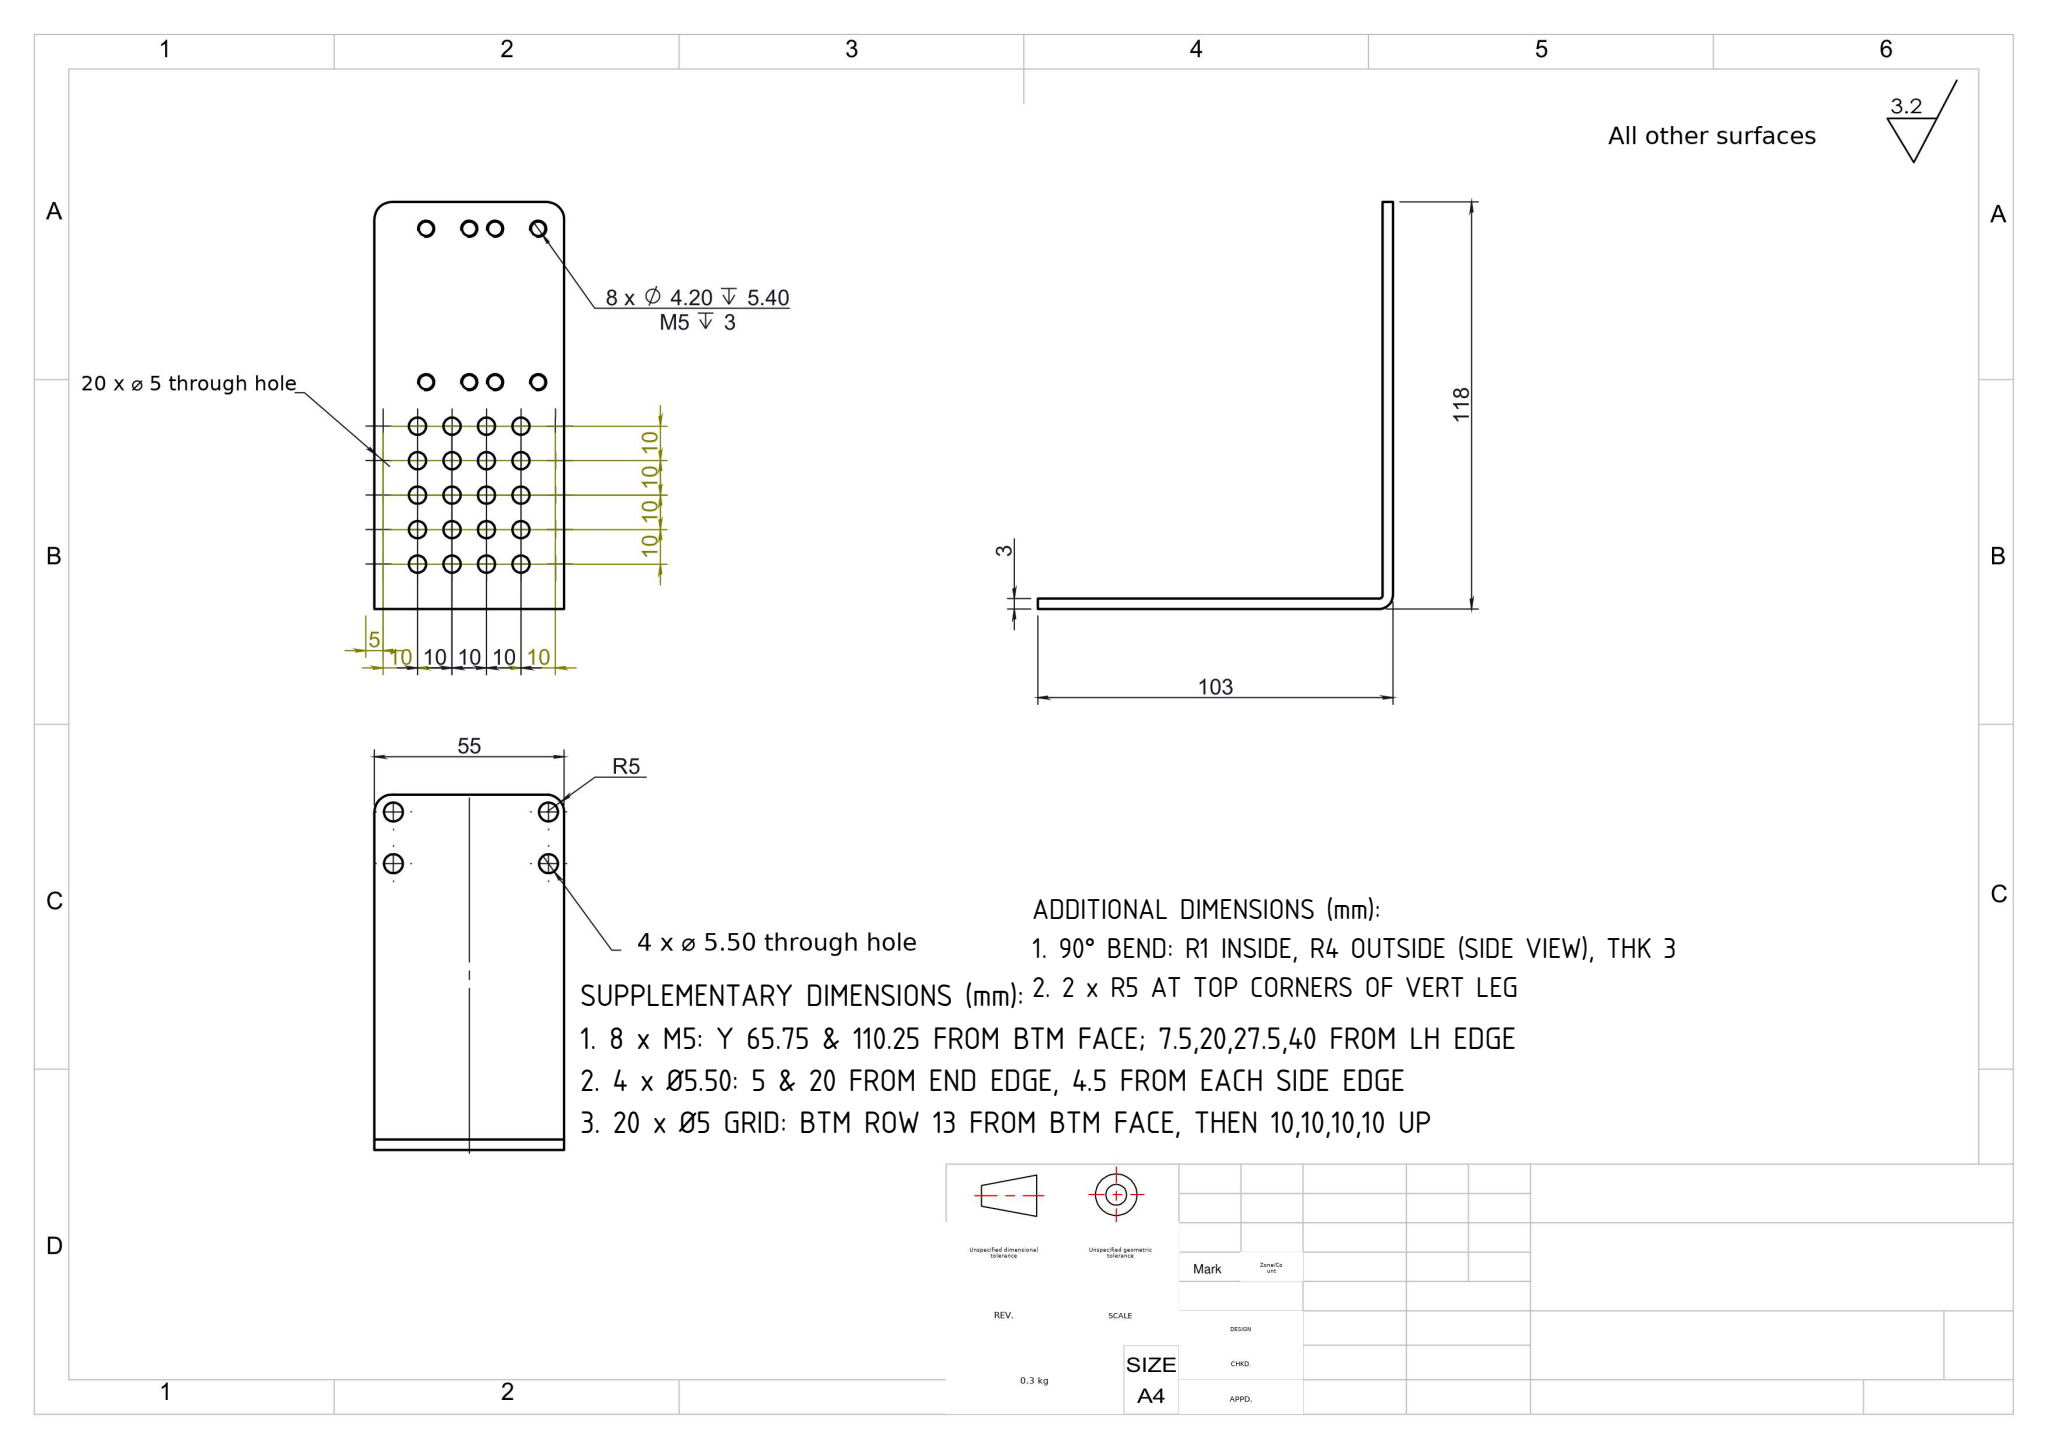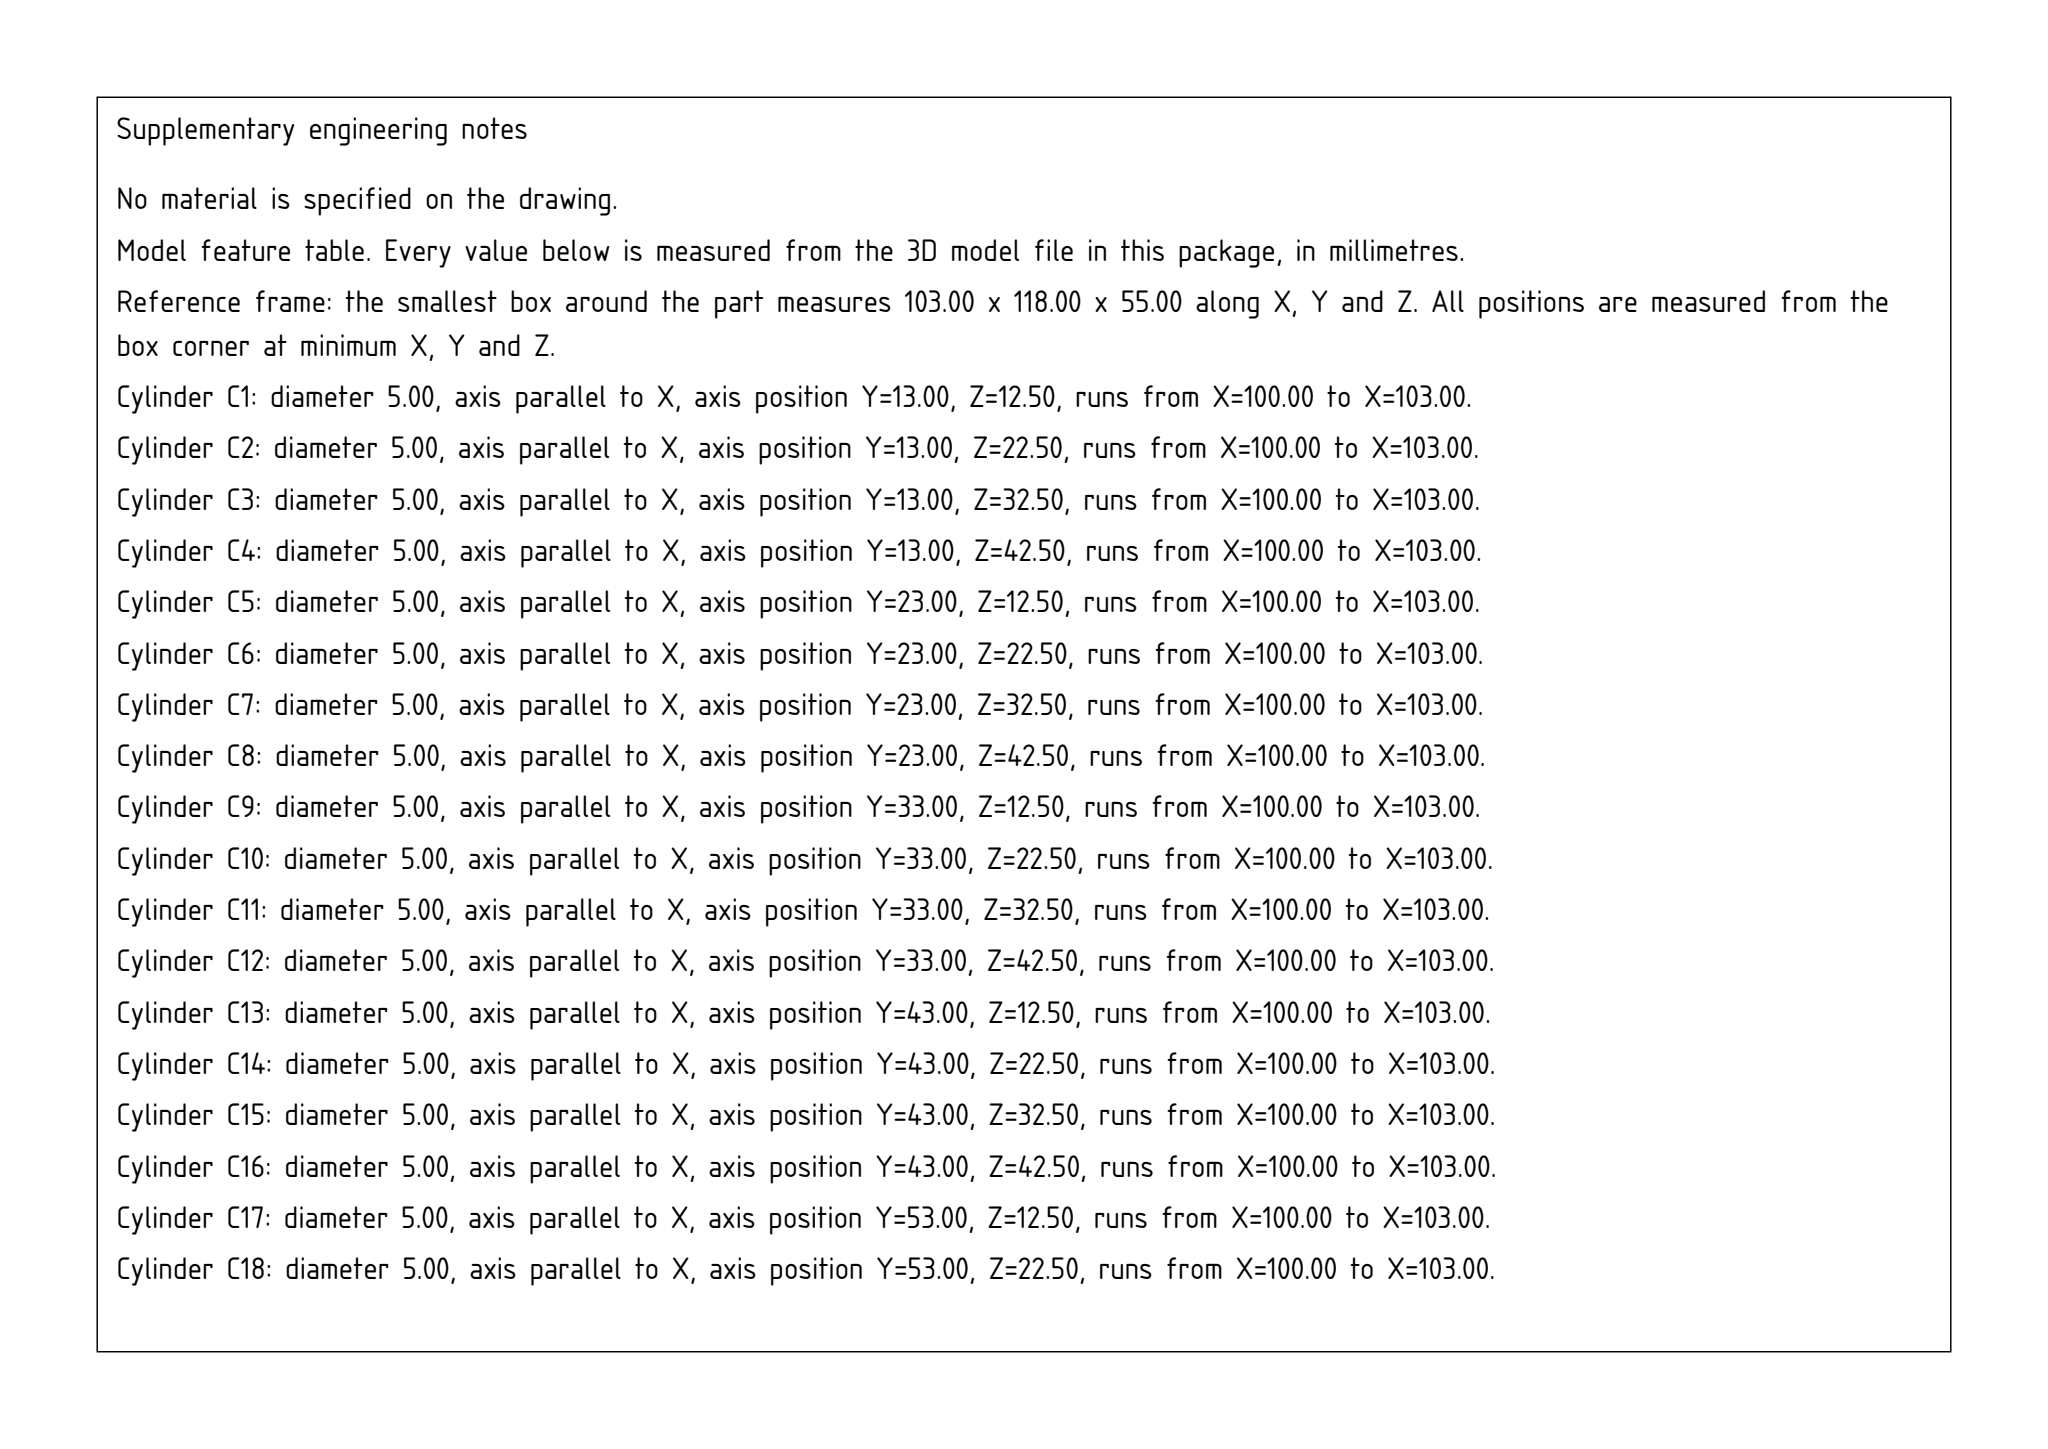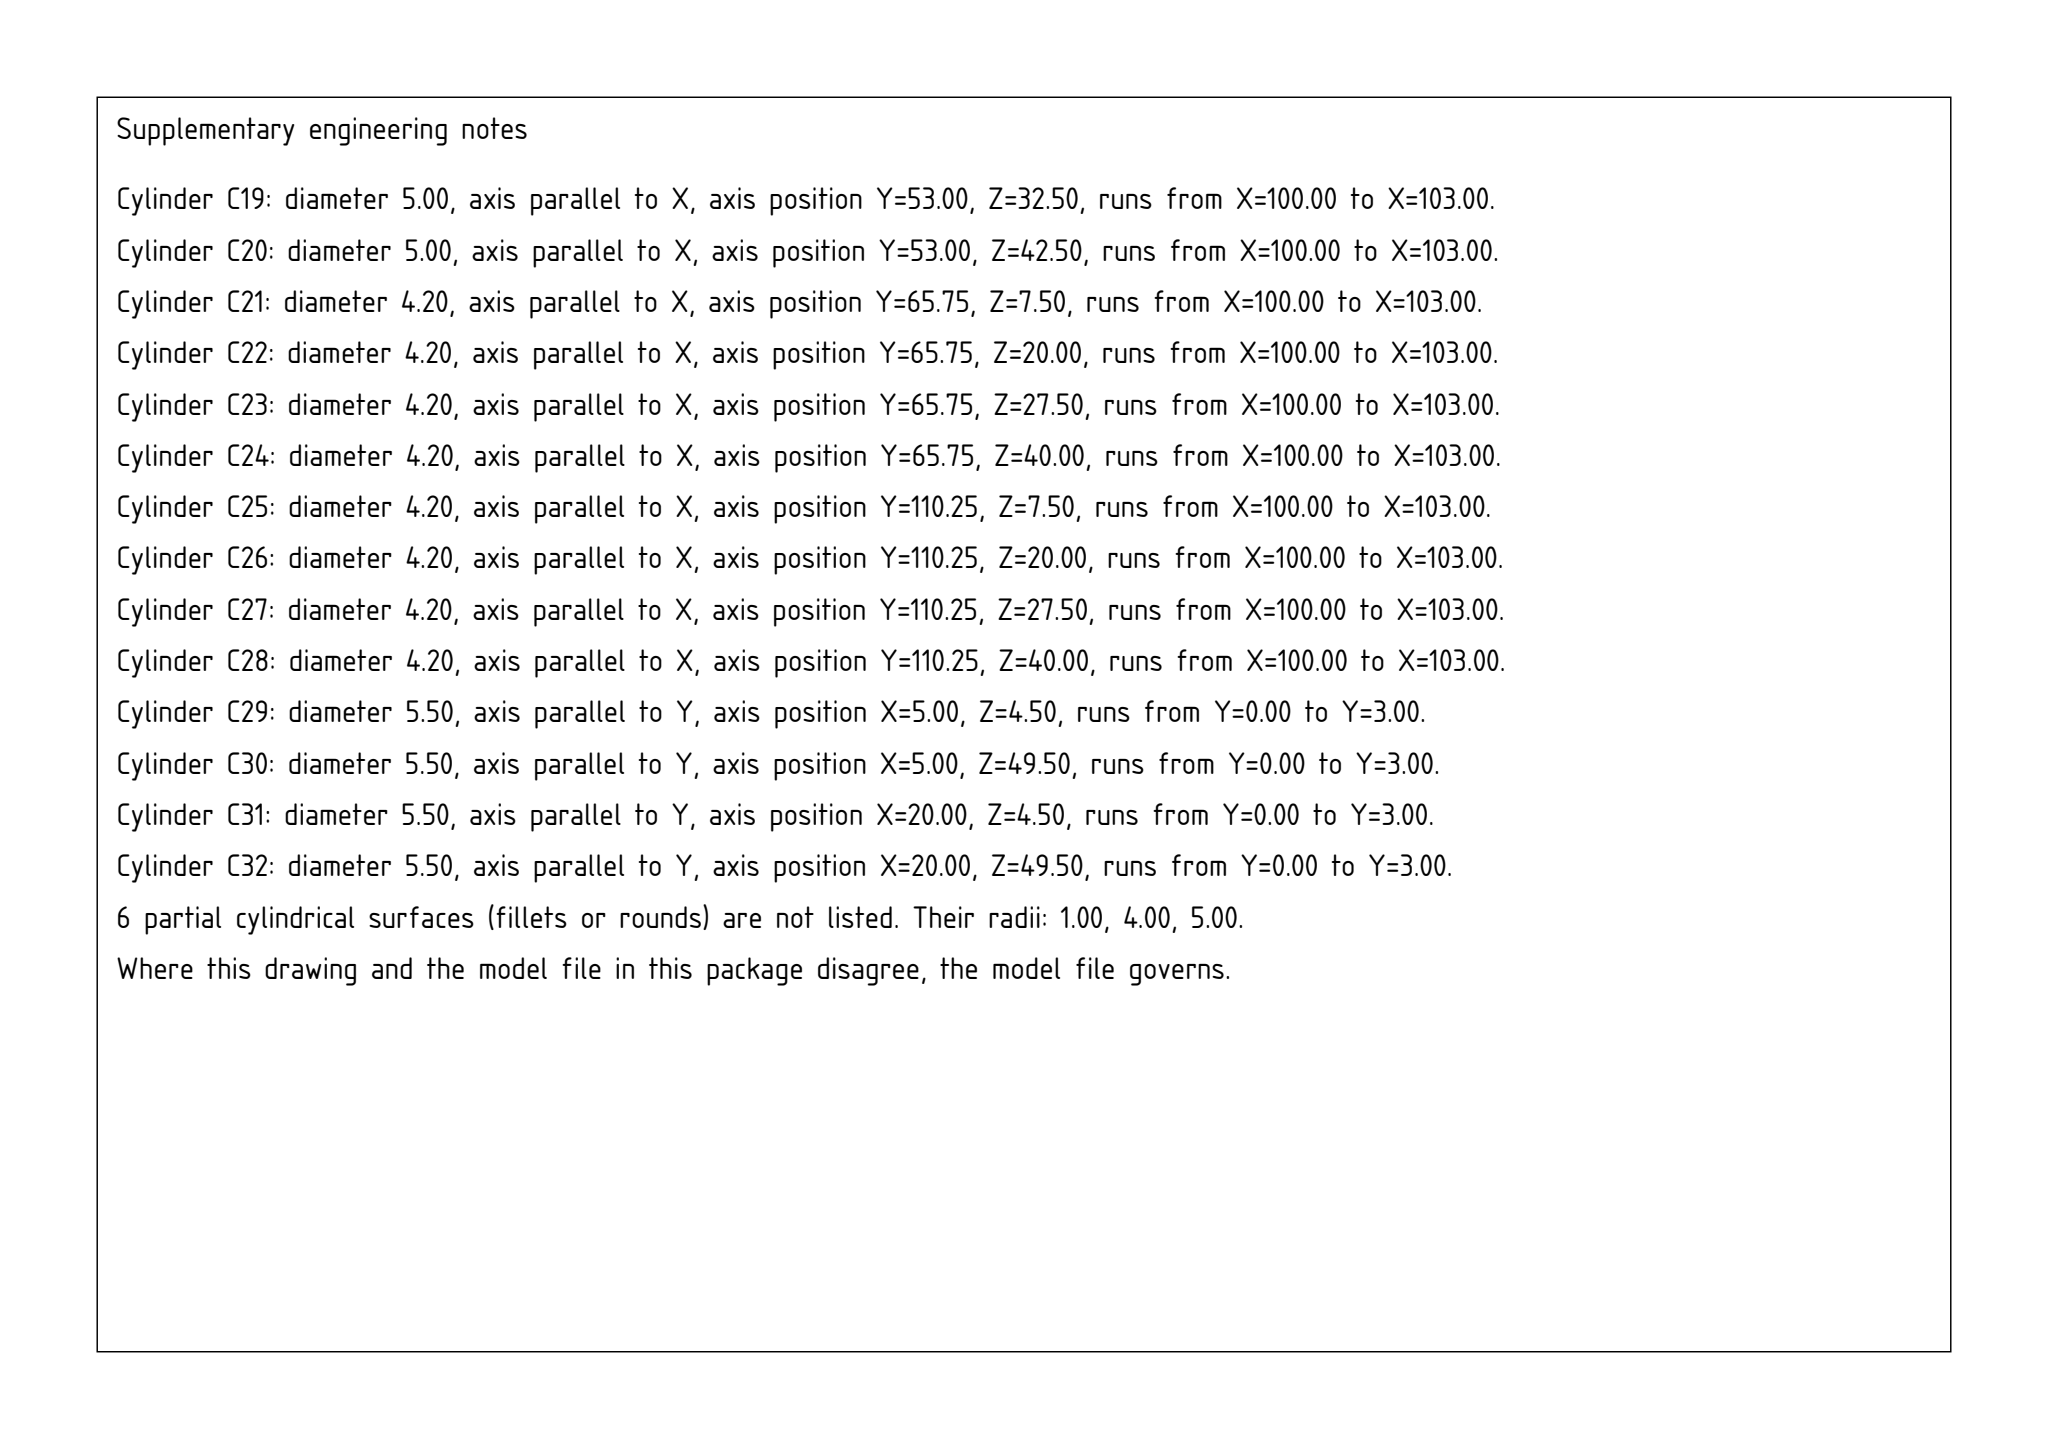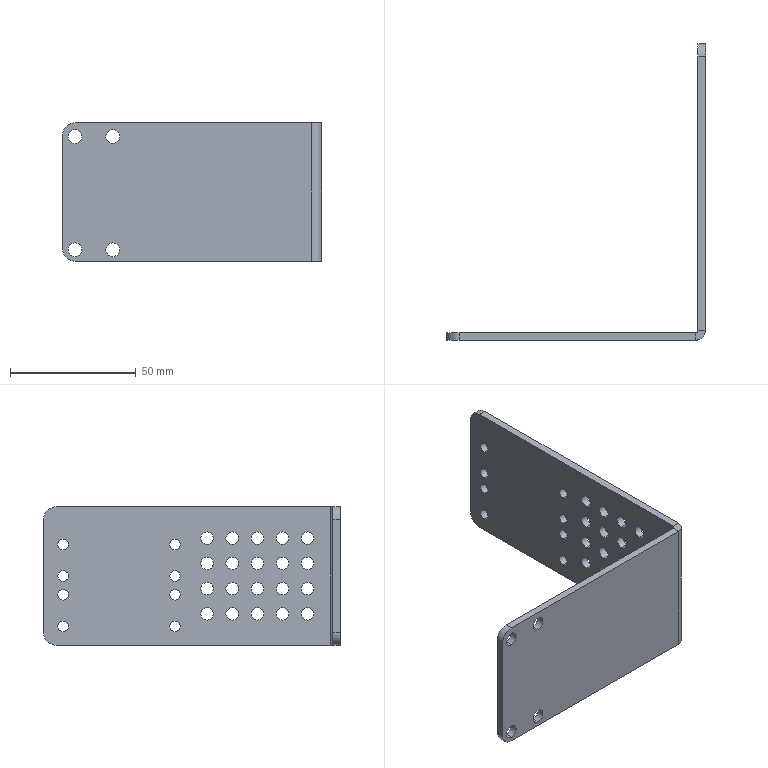Part | SolidWorks | mm | 1 solid | 82 faces | box 103 x 118 x 55 mm | volume 33933 mm3 | cylinder 70 | plane 12 | commonest cylinder face diameters 5 x40 4.2 x16 5.5 x8 10 x4 2 x1 8 x1